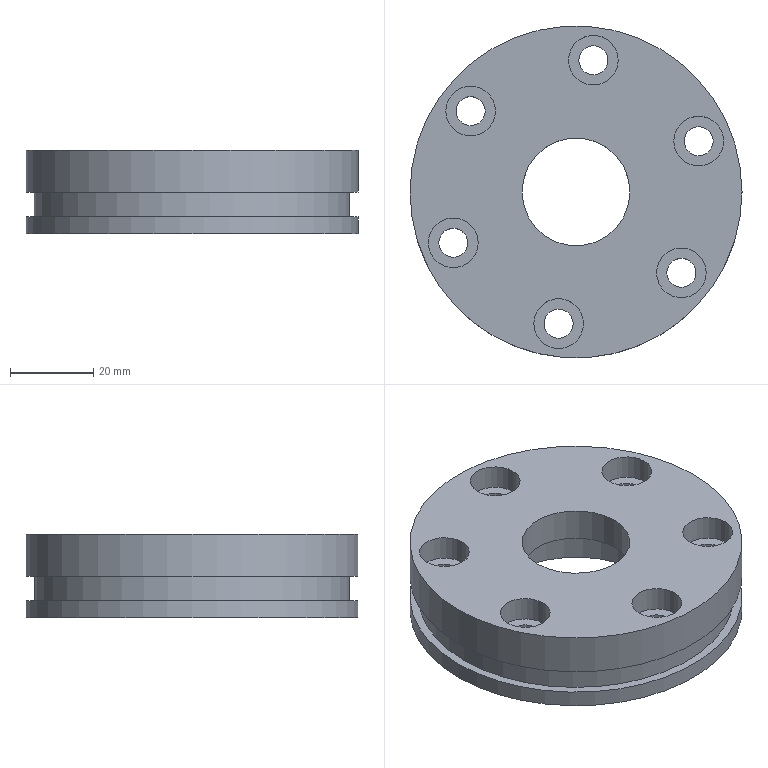Component | NX | CH3404_1-1 | 1 solid | 28 faces | volume 67792 mm3 | cylinder 17 | plane 11 | commonest cylinder face diameters 7 x6 12 x6 80 x2 44 x1 26 x1 76 x1